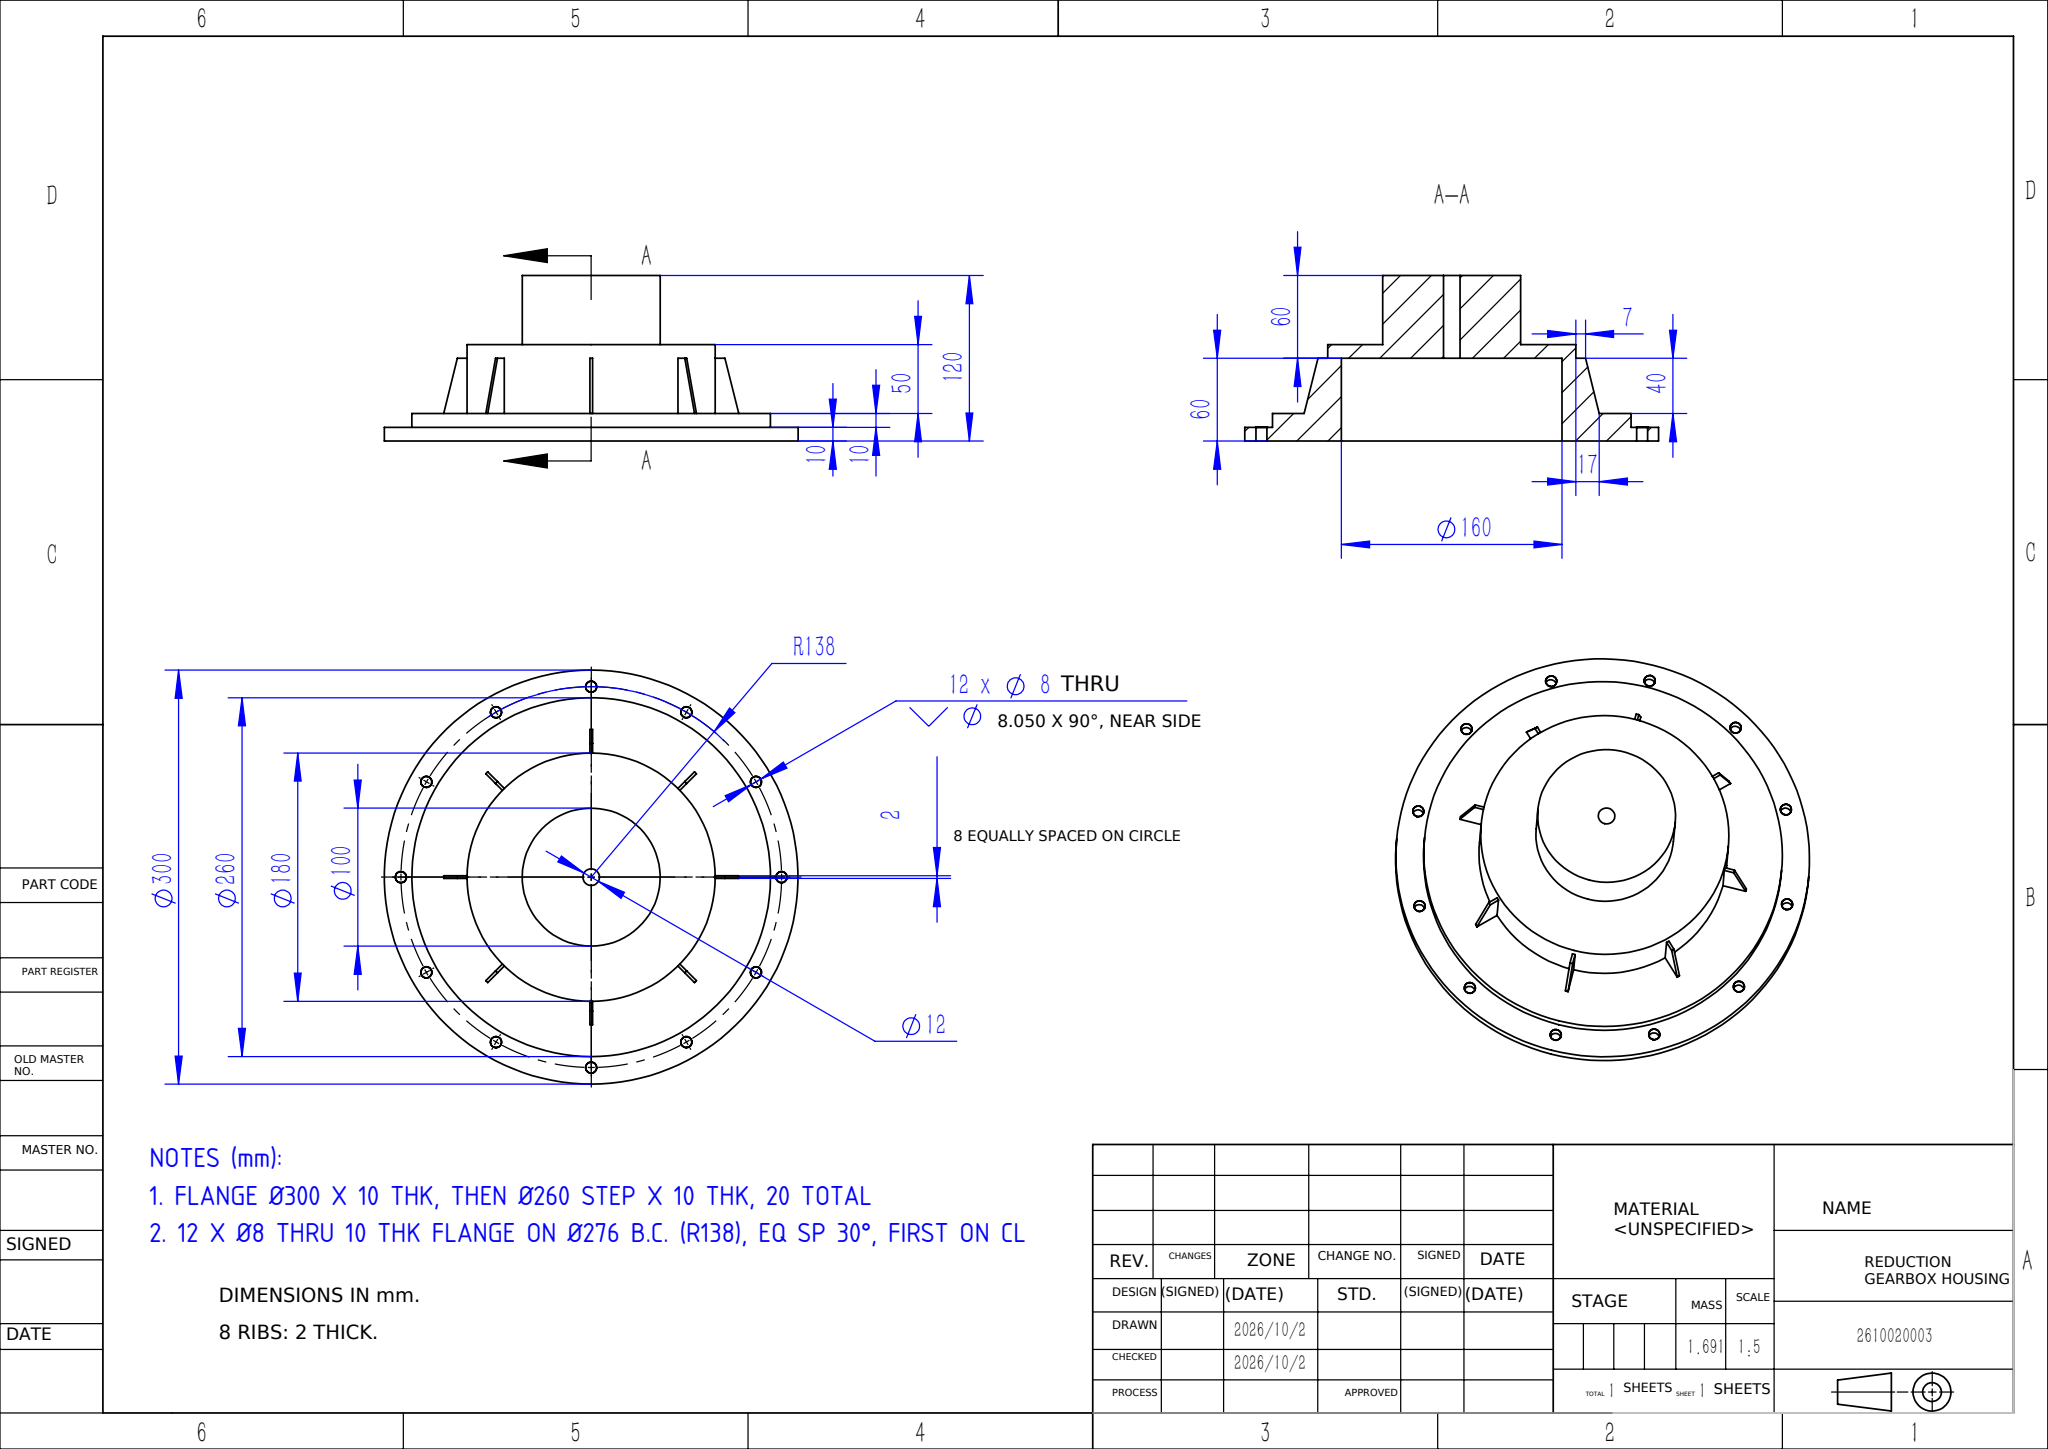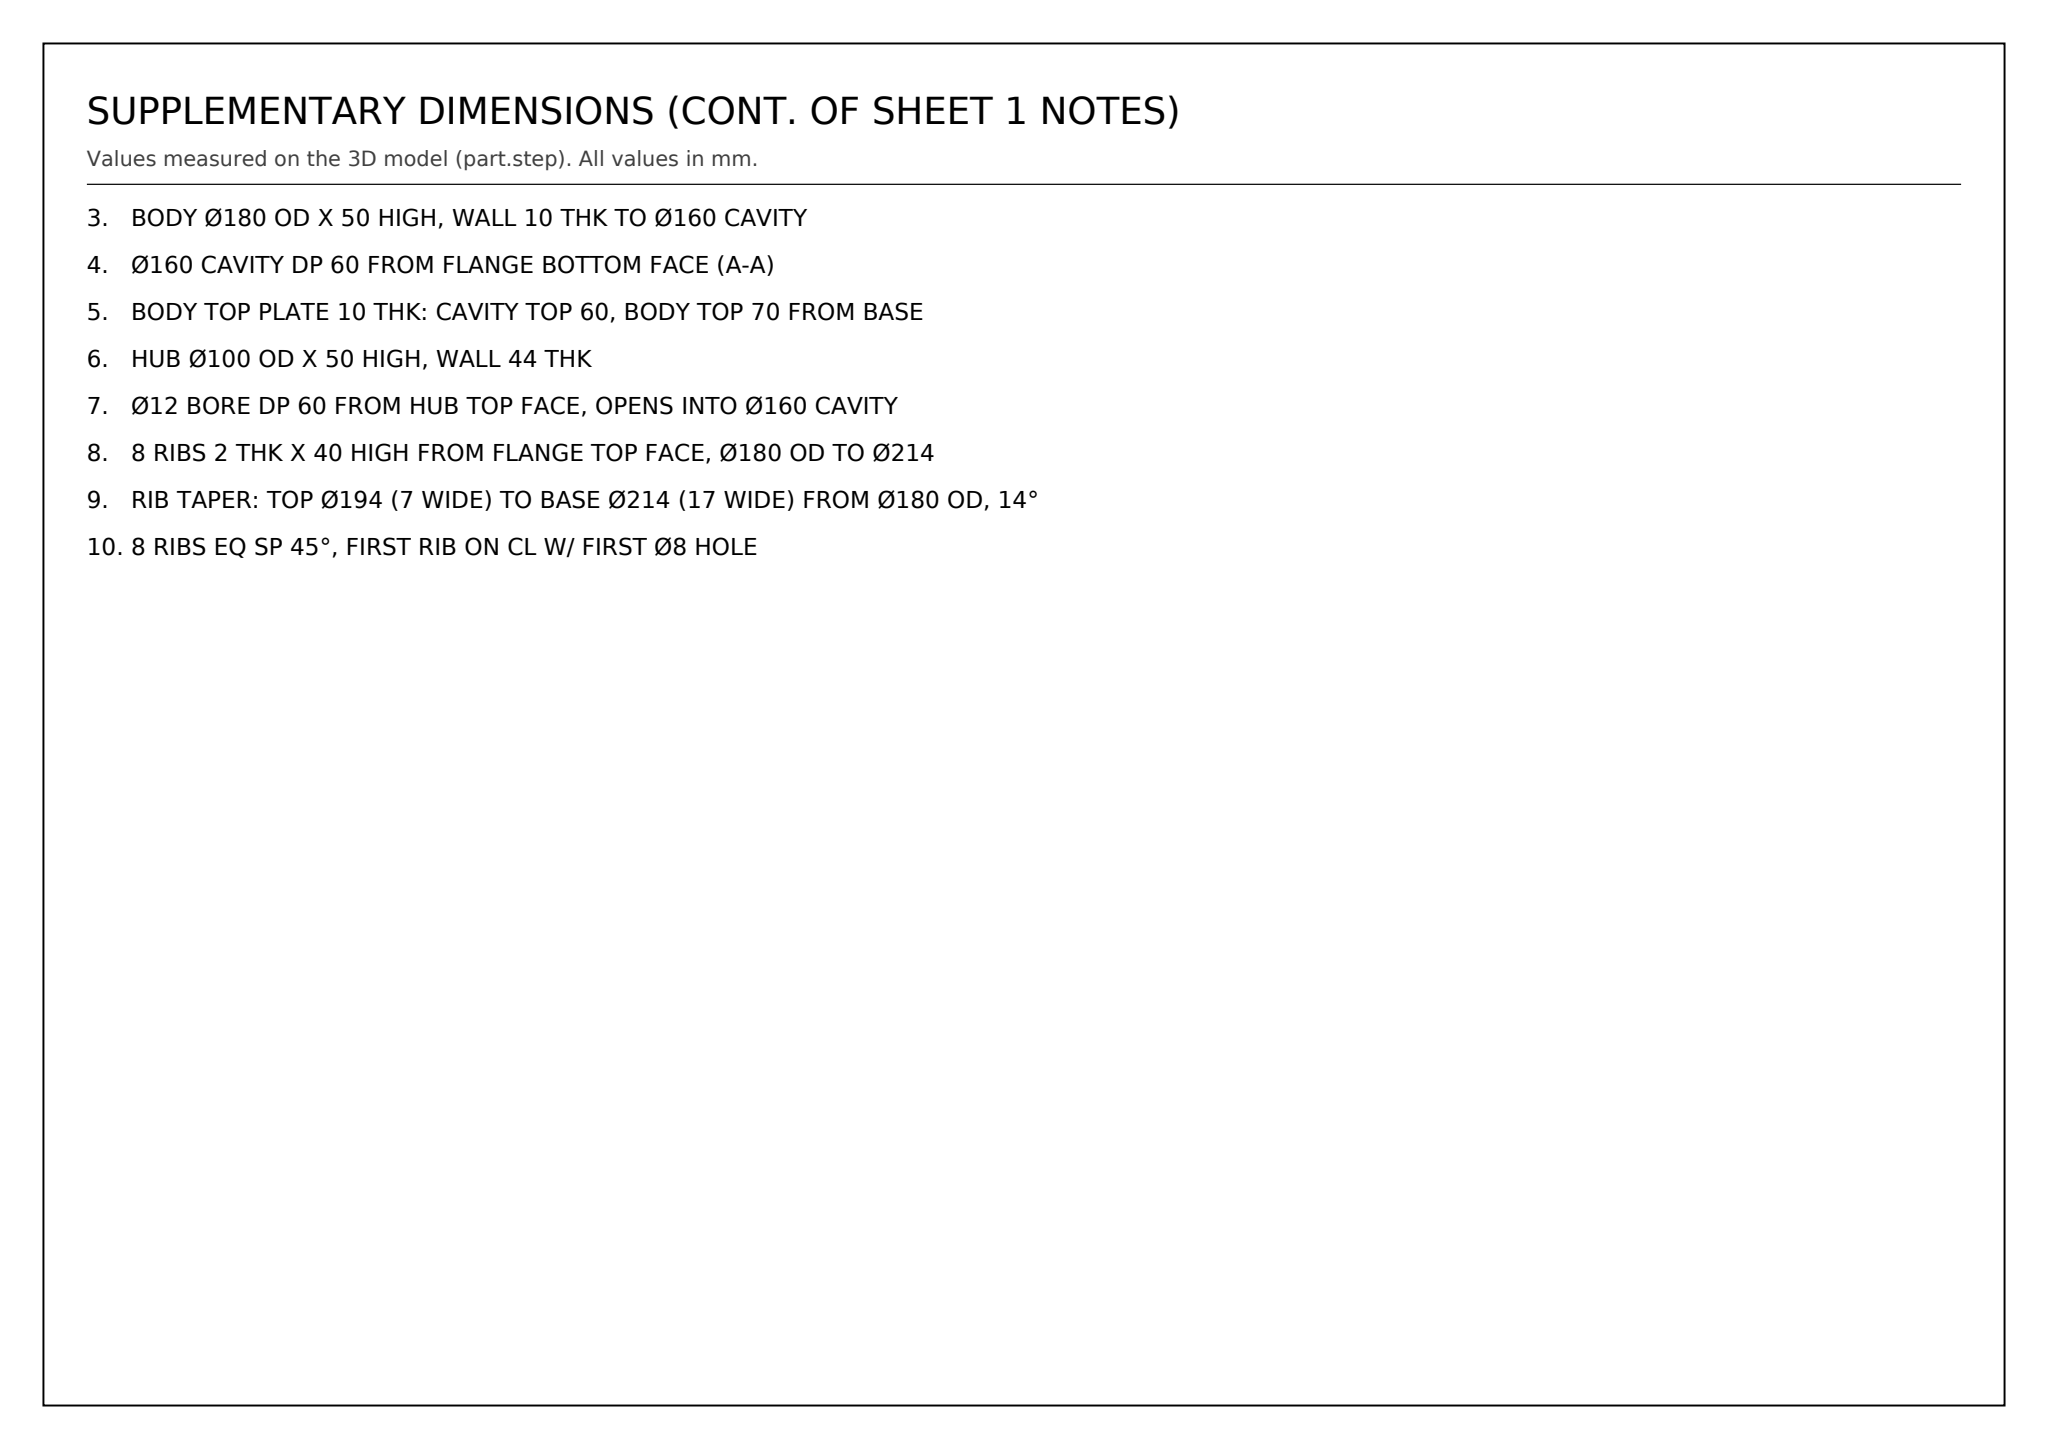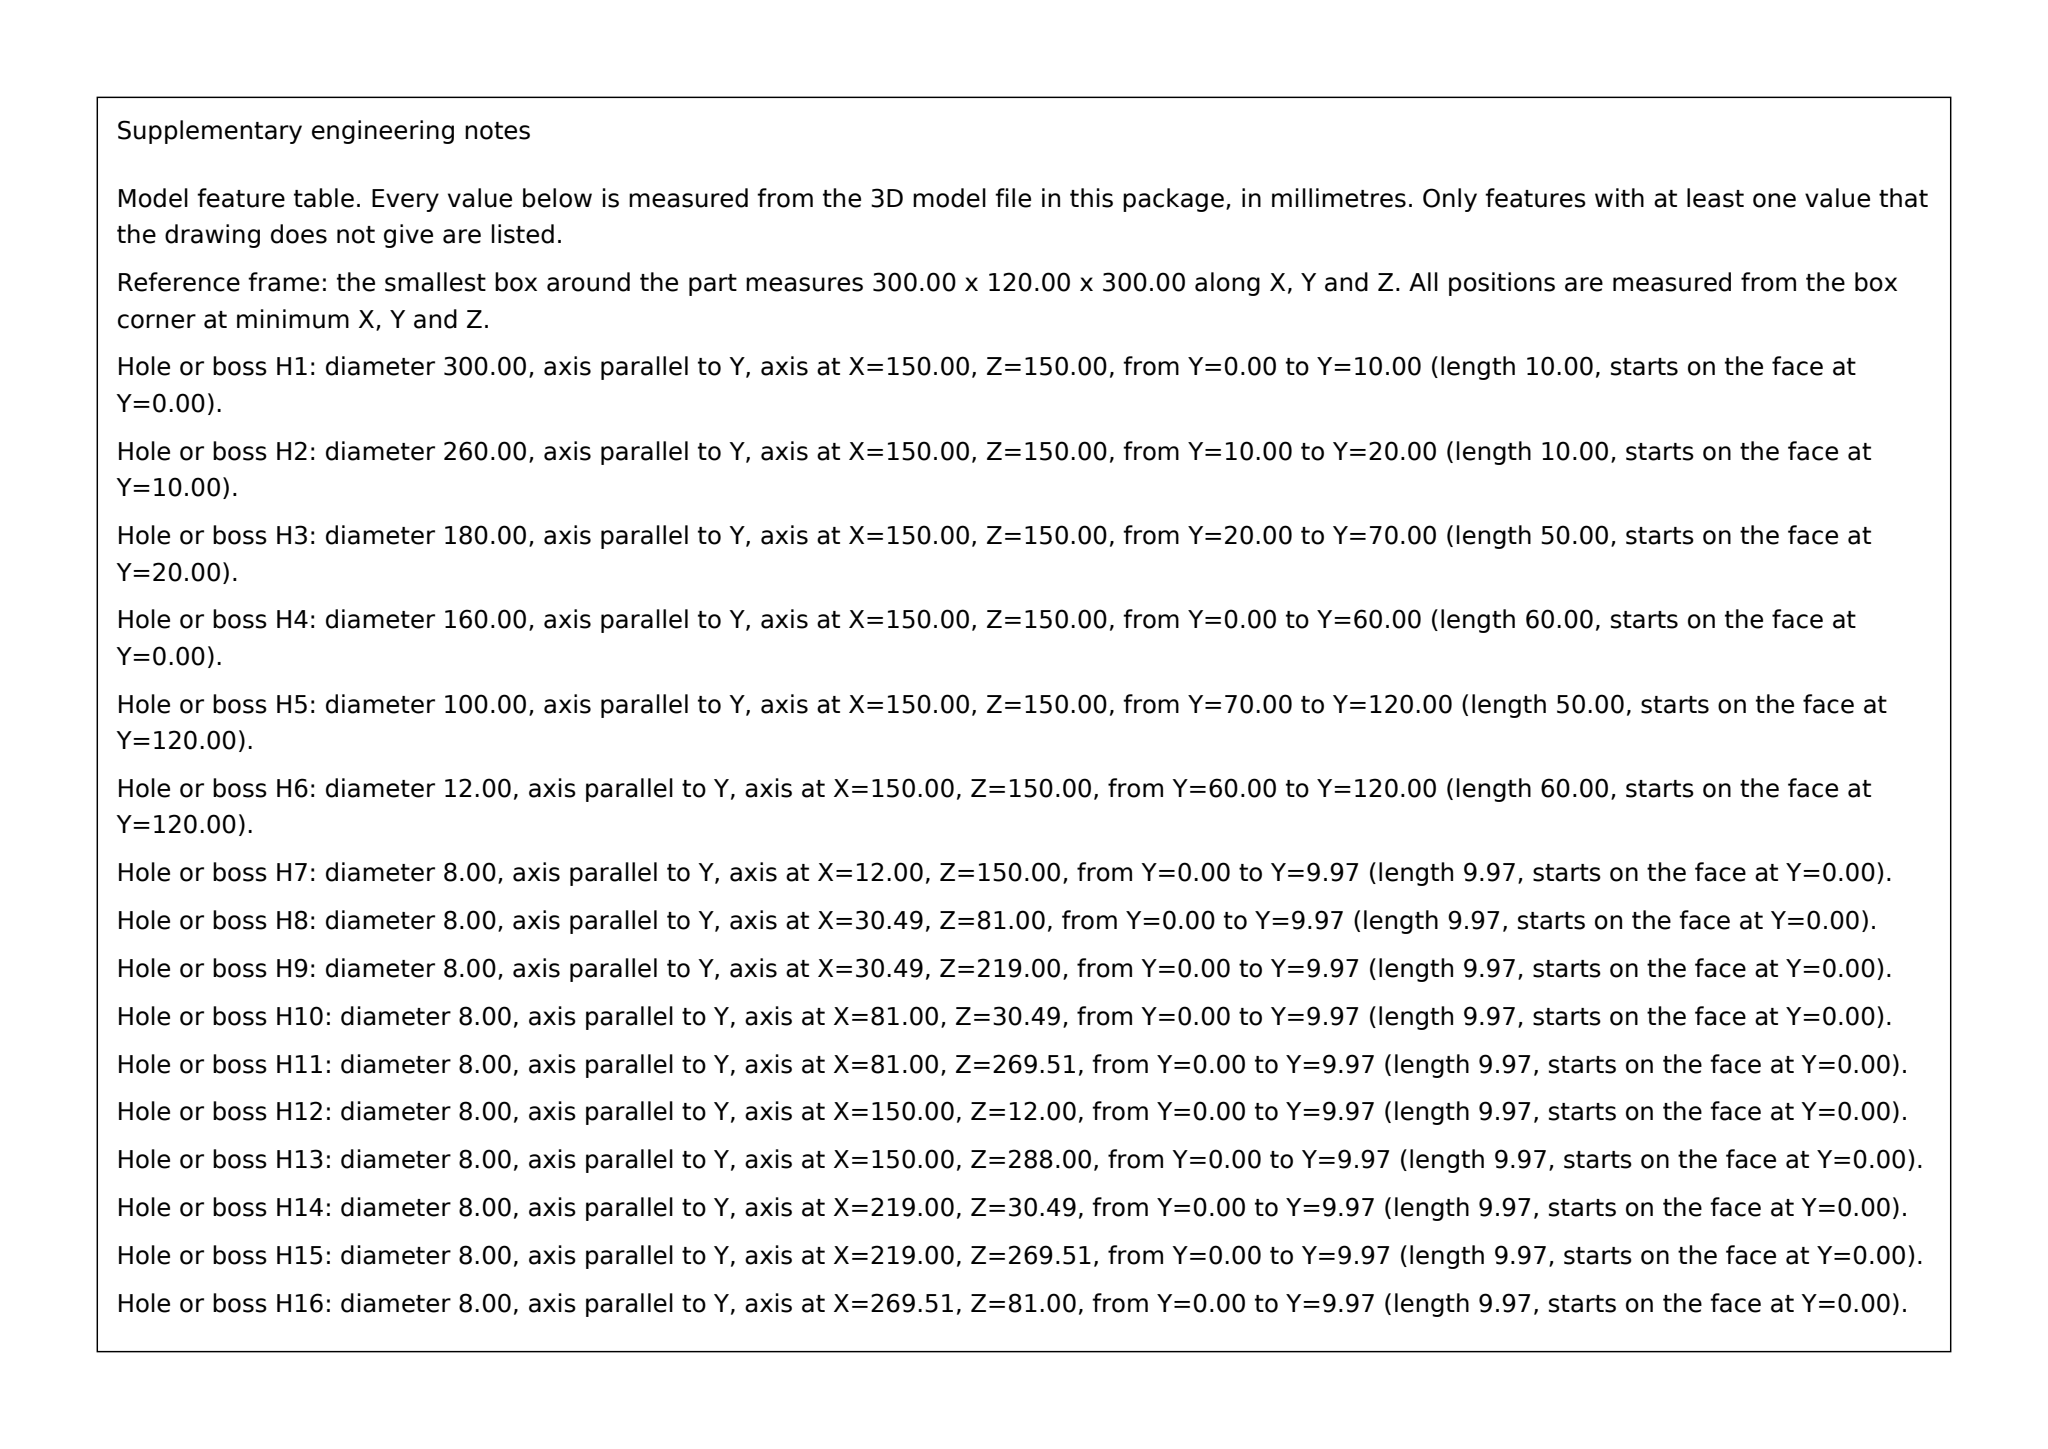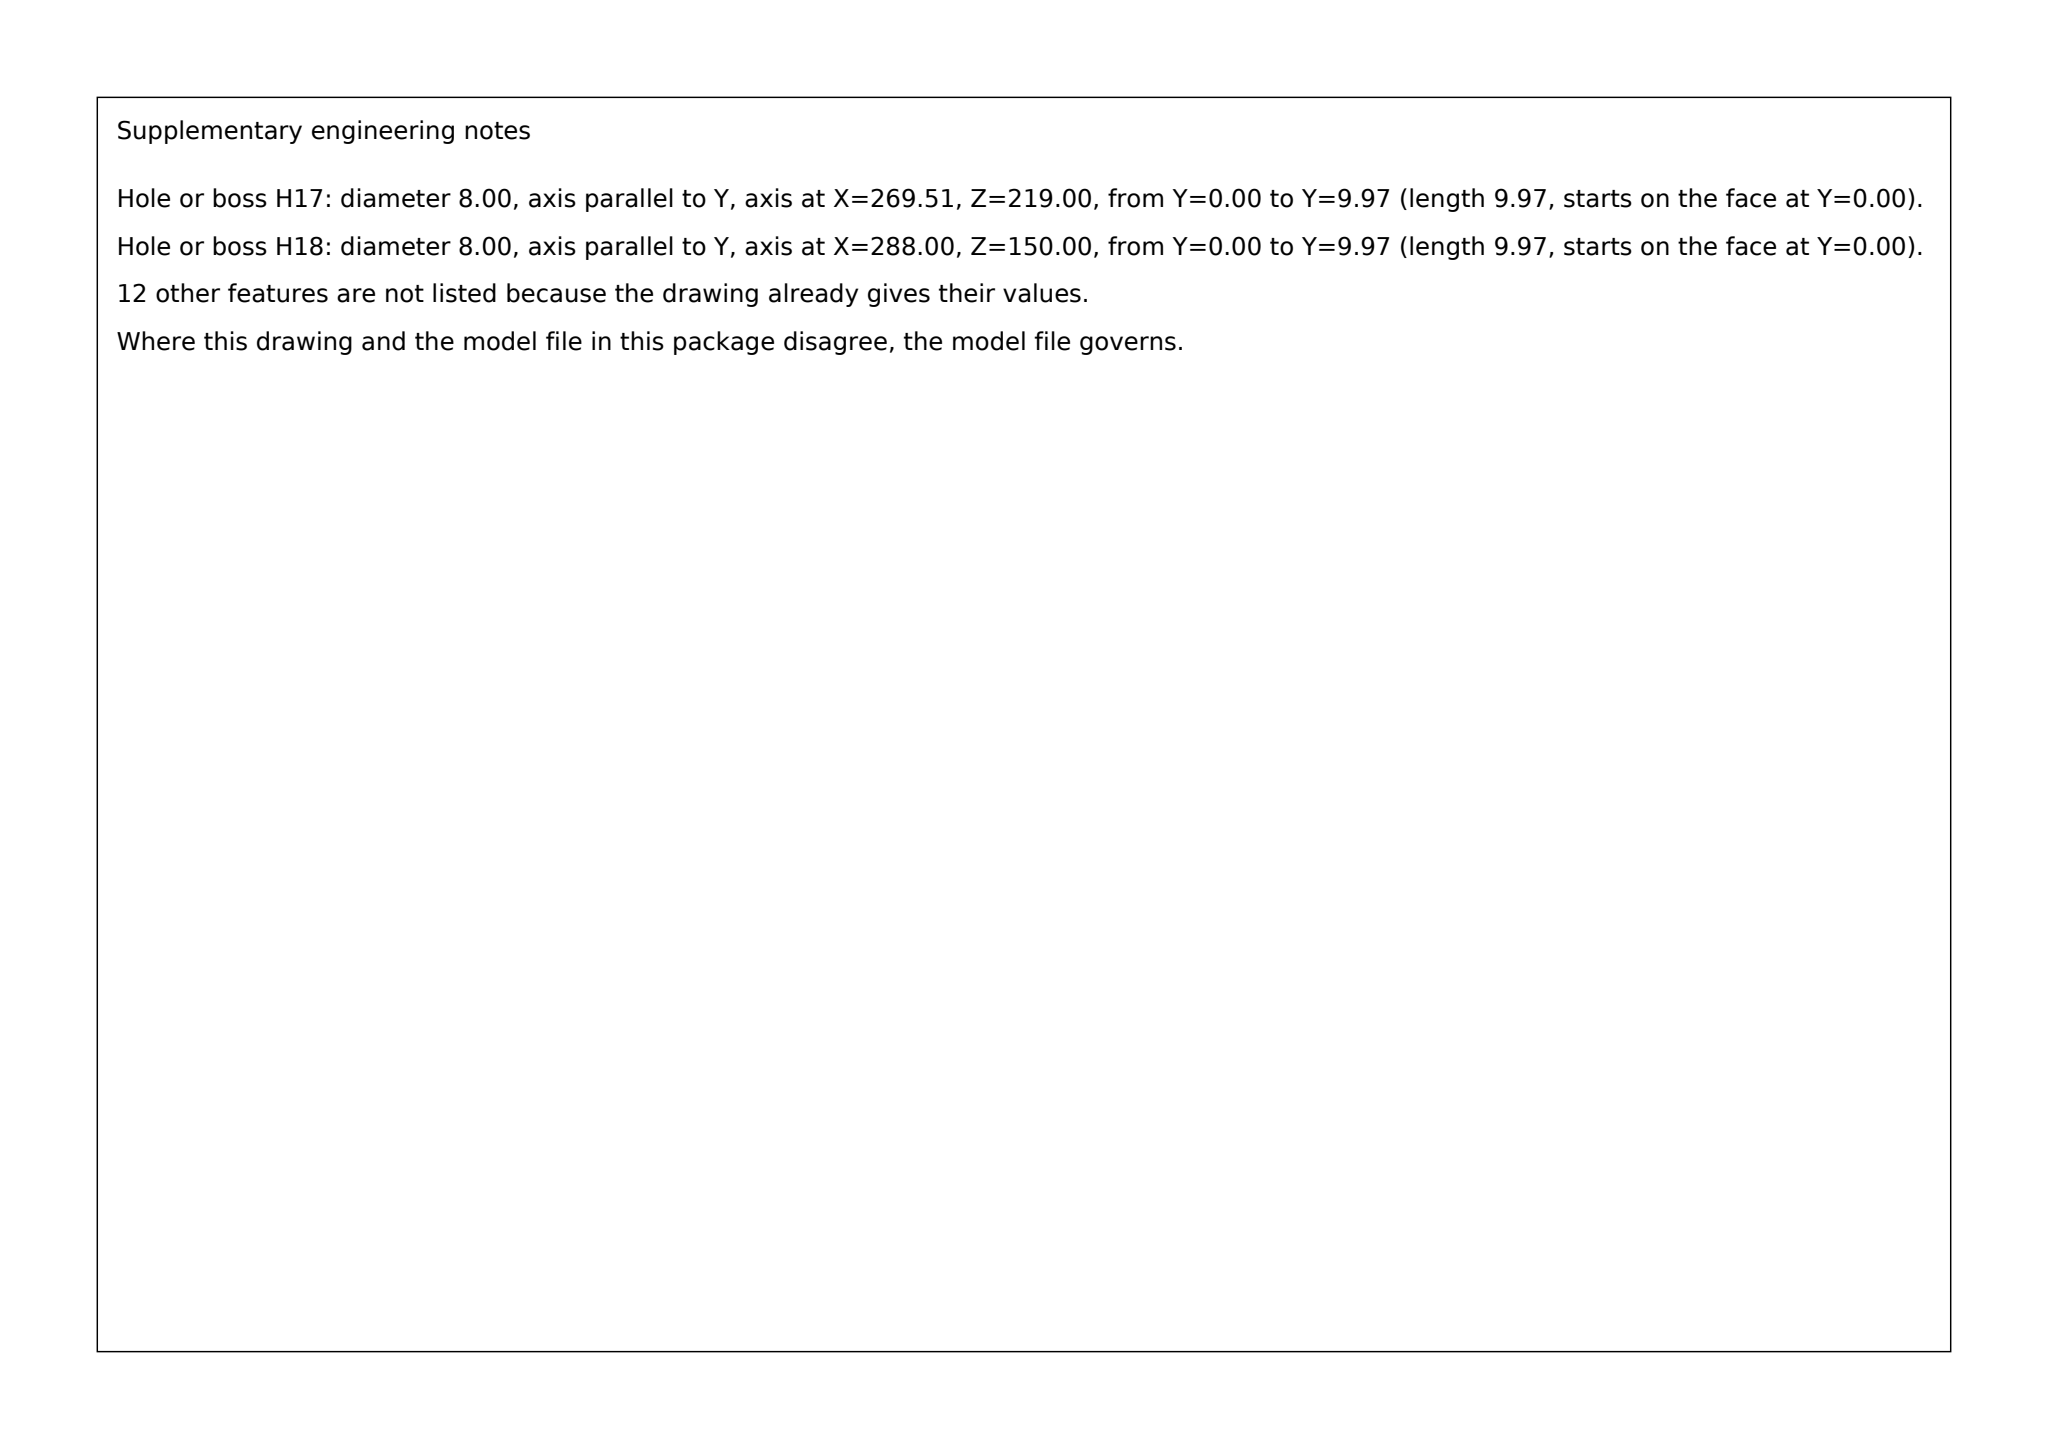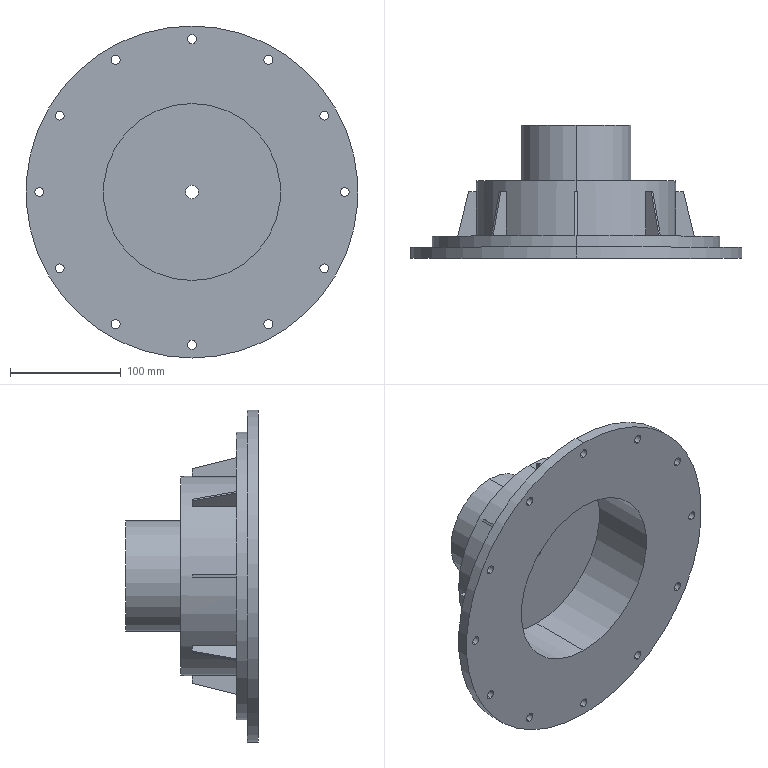Part | SolidWorks | mm | 1 solid | 98 faces | box 300 x 120 x 300 mm | volume 1691323 mm3 | plane 38 | cylinder 36 | cone 24 | commonest cylinder face diameters 8 x24 12 x2 160 x2 100 x2 180 x2 260 x2 300 x2
Drawing notes:
FLANGE Ø300 X 10 THK, THEN Ø260 STEP X 10 THK, 20 TOTAL | from the solid: cyl Ø300 len 10 (y=0-10), cyl Ø260 len 10 (y=10-20); planes y=0,10,20
12 X Ø8 THRU 10 THK FLANGE ON Ø276 B.C. (R138), EQ SP 30°, FIRST ON CL | from the solid: 12 cyls Ø8 axis y len 9.98 at R138 from (150,150); e.g. (12,150) on CL, (30.49,81), (81,30.49)
BODY Ø180 OD X 50 HIGH, WALL 10 THK TO Ø160 CAVITY | from the solid: cyl Ø180 len 50 (y=20-70) vs cyl Ø160 len 60 (y=0-60): (180-160)/2=10
Ø160 CAVITY DP 60 FROM FLANGE BOTTOM FACE (A-A) | from the solid: cyl Ø160 axis y at (150,150) len 60, y=0 to y=60; planes y=0 and y=60
BODY TOP PLATE 10 THK: CAVITY TOP 60, BODY TOP 70 FROM BASE | from the solid: planes y=60 (9 faces) and y=70 (1 face), base plane y=0
HUB Ø100 OD X 50 HIGH, WALL 44 THK | from the solid: cyl Ø100 len 50 (y=70 to 120), cyl Ø12 len 60: (100-12)/2=44
Ø12 BORE DP 60 FROM HUB TOP FACE, OPENS INTO Ø160 CAVITY | from the solid: cyl Ø12 axis y at (150,150) len 60, from y=120 to y=60; Ø160 cavity top plane y=60
8 RIBS 2 THK X 40 HIGH FROM FLANGE TOP FACE, Ø180 OD TO Ø214 | from the solid: rib faces at x=149/151 & z=149/151 (2 THK); flat tops y=60 over flange top y=20 = 40 high
RIB TAPER: TOP Ø194 (7 WIDE) TO BASE Ø214 (17 WIDE) FROM Ø180 OD, 14° | from the solid: rib top y=60 extends 7 from Ø180 (A-A 7), base y=20 extends 17 (A-A 17); 10/40 = 14.04°
8 RIBS EQ SP 45°, FIRST RIB ON CL W/ FIRST Ø8 HOLE | from the solid: rib side planes on x=150 and z=150 CLs (149/151 pairs), same CL as Ø8 hole at (150,12)
build123d program:
from build123d import *

# Parameters (mm, degrees)
SKETCH1_R                          = 150
BOSS_EXTRUDE1_DEPTH                = 10
SKETCH2_R                          = 130
BOSS_EXTRUDE2_DEPTH                = 10
SKETCH3_R                          = 90
BOSS_EXTRUDE3_DEPTH                = 50
SKETCH4_R                          = 50
BOSS_EXTRUDE4_DEPTH                = 50
SKETCH5_R                          = 80
CUT_EXTRUDE1_DEPTH                 = 60
BOSS_EXTRUDE8_DEPTH                = 1
CIRPATTERN1_COUNT                  = 8
SKETCH7_R                          = 6
CUT_EXTRUDE2_DEPTH                 = 244.721
F_8_0_8_DIAMETER_HOLE1_D           = 8
F_8_0_8_DIAMETER_HOLE1_CSINK_D     = 8.05
F_8_0_8_DIAMETER_HOLE1_CSINK_ANGLE = 90


with BuildPart() as part:
    # Sketch1 → Boss-Extrude1 (new body)
    with BuildSketch(Plane(origin=(0, 0, 0), x_dir=(1, 0, 0), z_dir=(0, 1, 0))):
        with Locations(Location((0, 0, 0), (0, 0, 270))):
            Circle(SKETCH1_R)
    extrude(amount=BOSS_EXTRUDE1_DEPTH)

    # Sketch2 → Boss-Extrude2 (add)
    with BuildSketch(Plane(origin=(0, 10, 0), x_dir=(1, 0, 0), z_dir=(0, 1, 0))):
        with Locations(Location((0, 0, 0), (0, 0, 270))):
            Circle(SKETCH2_R)
    extrude(amount=BOSS_EXTRUDE2_DEPTH)

    # Sketch3 → Boss-Extrude3 (add)
    with BuildSketch(Plane(origin=(0, 20, 0), x_dir=(1, 0, 0), z_dir=(0, 1, 0))):
        with Locations(Location((0, 0, 0), (0, 0, 270))):
            Circle(SKETCH3_R)
    extrude(amount=BOSS_EXTRUDE3_DEPTH)

    # Sketch4 → Boss-Extrude4 (add)
    with BuildSketch(Plane(origin=(0, 70, 0), x_dir=(1, 0, 0), z_dir=(0, 1, 0))):
        with Locations(Location((0, 0, 0), (0, 0, 270))):
            Circle(SKETCH4_R)
    extrude(amount=BOSS_EXTRUDE4_DEPTH)

    # Sketch5 → Cut-Extrude1 (cut)
    with BuildSketch(Plane.XZ):
        with Locations(Location((0, 0, 0), (0, 0, 270))):
            Circle(SKETCH5_R)
    extrude(amount=-CUT_EXTRUDE1_DEPTH, mode=Mode.SUBTRACT)

    # Sketch6 → Boss-Extrude8 (add, symmetric)
    with BuildSketch(Plane(origin=(0, 0, 0), x_dir=(0, 0, -1), z_dir=(1, 0, 0))):
        Polygon((-87, 60), (-97, 60), (-107, 20), (-87, 20), align=None)
    boss_extrude8 = extrude(amount=BOSS_EXTRUDE8_DEPTH, both=True)

    # CirPattern1: Boss-Extrude8 ×8 about axis
    cirpattern1_axis = Axis((0, 0, 0), (0, 1, 0))
    for i in range(1, CIRPATTERN1_COUNT):
        add(boss_extrude8.rotate(cirpattern1_axis, i * 360 / CIRPATTERN1_COUNT))

    # Sketch7 → Cut-Extrude2 (cut, through all)
    with BuildSketch(Plane(origin=(0, 120, 0), x_dir=(1, 0, 0), z_dir=(0, 1, 0))):
        with Locations(Location((0, 0, 0), (0, 0, 270))):
            Circle(SKETCH7_R)
    extrude(amount=-CUT_EXTRUDE2_DEPTH, mode=Mode.SUBTRACT)

    # 8.0 _8_ Diameter Hole1 (through all)
    with Locations(Plane(origin=(0, 10, 0), x_dir=(1, 0, 0), z_dir=(0, 1, 0))):
        with Locations((-138, 0), (-119.512, 69), (-69, 119.512), (0, 138), (69, 119.512), (119.512, 69), (138, 0), (119.512, -69), (69, -119.512), (0, -138), (-69, -119.512), (-119.512, -69)):
            CounterSinkHole(F_8_0_8_DIAMETER_HOLE1_D / 2, F_8_0_8_DIAMETER_HOLE1_CSINK_D / 2, counter_sink_angle=F_8_0_8_DIAMETER_HOLE1_CSINK_ANGLE)


solid = part.part